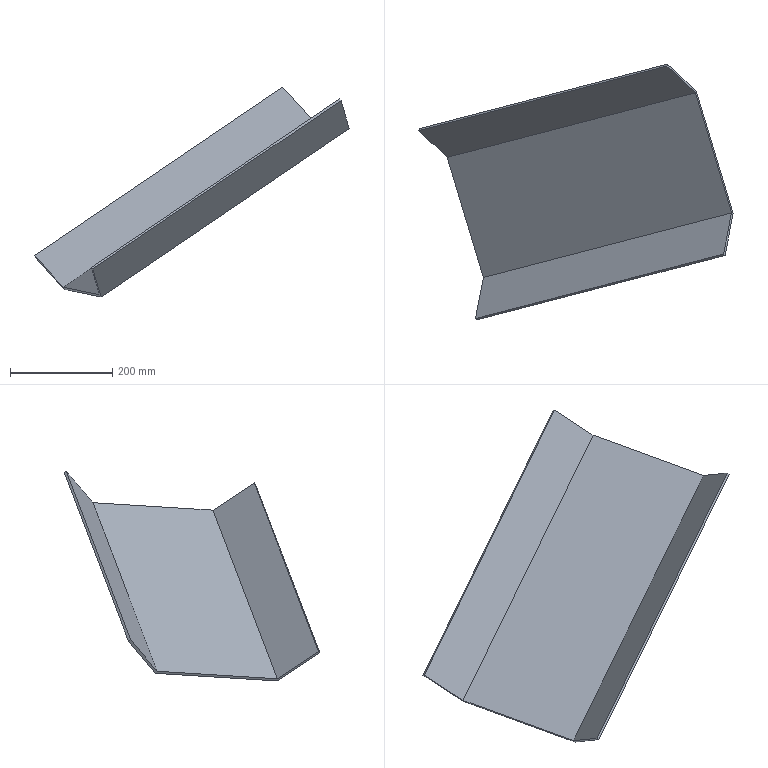Component | SolidWorks | CrusherFrameBaffle-1 | 1 solid | 10 faces | box 614.71 x 499.76 x 410.48 mm | volume 1337574 mm3 | plane 10
build123d program:
from build123d import *

# Parameters (mm, degrees)
EXTRUDE_THIN1_DEPTH = 600


with BuildPart() as part:
    # Sketch1 → Extrude-Thin1 (new body)
    with BuildSketch(Plane.XY):
        Polygon((70.711, -70.711), (0, 0), (0, 250), (70.711, 320.711), (74.246, 317.175), (5, 247.929), (5, 2.071), (74.246, -67.175), align=None)
    extrude(amount=EXTRUDE_THIN1_DEPTH)


solid = part.part

# Placed as in the assembly
solid = solid.moved(Location((-188.681, -31.644, -552.552), (-20.862, 53.982, -150.678)))
STEP:
#1=CARTESIAN_POINT('',(-4.718,-10.616,-22.172));
#2=VERTEX_POINT('',#1);
#3=CARTESIAN_POINT('',(-5.331,-13.784,-20.063));
#4=VERTEX_POINT('',#3);
#5=CARTESIAN_POINT('',(-4.705,-10.549,-22.217));
#6=DIRECTION('',(-0.1589,-0.8218,0.5471));
#7=VECTOR('',#6,39.37);
#8=LINE('',#5,#7);
#9=EDGE_CURVE('',#2,#4,#8,.T.);
#10=ORIENTED_EDGE('',*,*,#9,.T.);
#11=CARTESIAN_POINT('',(13.775,-8.838,-7.083));
#12=VERTEX_POINT('',#11);
#13=CARTESIAN_POINT('',(13.775,-8.838,-7.083));
#14=DIRECTION('',(-0.8088,-0.2094,-0.5495));
#15=VECTOR('',#14,39.37);
#16=LINE('',#13,#15);
#17=EDGE_CURVE('',#12,#4,#16,.T.);
#18=ORIENTED_EDGE('',*,*,#17,.F.);
#19=CARTESIAN_POINT('',(14.388,-5.669,-9.192));
#20=VERTEX_POINT('',#19);
#21=CARTESIAN_POINT('',(14.401,-5.602,-9.237));
#22=DIRECTION('',(-0.1589,-0.8218,0.5471));
#23=VECTOR('',#22,39.37);
#24=LINE('',#21,#23);
#25=EDGE_CURVE('',#20,#12,#24,.T.);
#26=ORIENTED_EDGE('',*,*,#25,.F.);
#27=CARTESIAN_POINT('',(14.388,-5.669,-9.192));
#28=DIRECTION('',(-0.8088,-0.2094,-0.5495));
#29=VECTOR('',#28,39.37);
#30=LINE('',#27,#29);
#31=EDGE_CURVE('',#20,#2,#30,.T.);
#32=ORIENTED_EDGE('',*,*,#31,.T.);
#33=EDGE_LOOP('',(#10,#18,#26,#32));
#34=FACE_OUTER_BOUND('',#33,.T.);
#35=CARTESIAN_POINT('',(14.401,-5.602,-9.237));
#36=DIRECTION('',(0.5662,-0.5298,-0.6315));
#37=DIRECTION('',(0.1589,0.8218,-0.5471));
#38=AXIS2_PLACEMENT_3D('',#35,#36,#37);
#39=PLANE('',#38);
#40=ADVANCED_FACE('',(#34),#39,.F.);
#41=CARTESIAN_POINT('',(-5.22,-13.889,-20.187));
#42=VERTEX_POINT('',#41);
#43=CARTESIAN_POINT('',(-5.22,-13.889,-20.187));
#44=DIRECTION('',(-0.5662,0.5298,0.6315));
#45=VECTOR('',#44,39.37);
#46=LINE('',#43,#45);
#47=EDGE_CURVE('',#42,#4,#46,.T.);
#48=ORIENTED_EDGE('',*,*,#47,.F.);
#49=CARTESIAN_POINT('',(13.887,-8.942,-7.207));
#50=VERTEX_POINT('',#49);
#51=CARTESIAN_POINT('',(13.887,-8.942,-7.207));
#52=DIRECTION('',(-0.8088,-0.2094,-0.5495));
#53=VECTOR('',#52,39.37);
#54=LINE('',#51,#53);
#55=EDGE_CURVE('',#50,#42,#54,.T.);
#56=ORIENTED_EDGE('',*,*,#55,.F.);
#57=CARTESIAN_POINT('',(13.887,-8.942,-7.207));
#58=DIRECTION('',(-0.5662,0.5298,0.6315));
#59=VECTOR('',#58,39.37);
#60=LINE('',#57,#59);
#61=EDGE_CURVE('',#50,#12,#60,.T.);
#62=ORIENTED_EDGE('',*,*,#61,.T.);
#63=ORIENTED_EDGE('',*,*,#17,.T.);
#64=EDGE_LOOP('',(#48,#56,#62,#63));
#65=FACE_OUTER_BOUND('',#64,.T.);
#66=CARTESIAN_POINT('',(13.887,-8.942,-7.207));
#67=DIRECTION('',(-0.1589,-0.8218,0.5471));
#68=DIRECTION('',(0.5662,-0.5298,-0.6315));
#69=AXIS2_PLACEMENT_3D('',#66,#67,#68);
#70=PLANE('',#69);
#71=ADVANCED_FACE('',(#65),#70,.T.);
#72=CARTESIAN_POINT('',(-4.594,-10.653,-22.341));
#73=VERTEX_POINT('',#72);
#74=CARTESIAN_POINT('',(-4.594,-10.653,-22.341));
#75=DIRECTION('',(-0.1589,-0.8218,0.5471));
#76=VECTOR('',#75,39.37);
#77=LINE('',#74,#76);
#78=EDGE_CURVE('',#73,#42,#77,.T.);
#79=ORIENTED_EDGE('',*,*,#78,.F.);
#80=CARTESIAN_POINT('',(14.512,-5.706,-9.361));
#81=VERTEX_POINT('',#80);
#82=CARTESIAN_POINT('',(14.512,-5.706,-9.361));
#83=DIRECTION('',(-0.8088,-0.2094,-0.5495));
#84=VECTOR('',#83,39.37);
#85=LINE('',#82,#84);
#86=EDGE_CURVE('',#81,#73,#85,.T.);
#87=ORIENTED_EDGE('',*,*,#86,.F.);
#88=CARTESIAN_POINT('',(14.512,-5.706,-9.361));
#89=DIRECTION('',(-0.1589,-0.8218,0.5471));
#90=VECTOR('',#89,39.37);
#91=LINE('',#88,#90);
#92=EDGE_CURVE('',#81,#50,#91,.T.);
#93=ORIENTED_EDGE('',*,*,#92,.T.);
#94=ORIENTED_EDGE('',*,*,#55,.T.);
#95=EDGE_LOOP('',(#79,#87,#93,#94));
#96=FACE_OUTER_BOUND('',#95,.T.);
#97=CARTESIAN_POINT('',(14.512,-5.706,-9.361));
#98=DIRECTION('',(0.5662,-0.5298,-0.6315));
#99=DIRECTION('',(0.1589,0.8218,-0.5471));
#100=AXIS2_PLACEMENT_3D('',#97,#98,#99);
#101=PLANE('',#100);
#102=ADVANCED_FACE('',(#96),#101,.T.);
#103=CARTESIAN_POINT('',(-7.428,-1.246,-21.754));
#104=VERTEX_POINT('',#103);
#105=CARTESIAN_POINT('',(-7.428,-1.246,-21.754));
#106=DIRECTION('',(0.288,-0.9558,-0.05964));
#107=VECTOR('',#106,39.37);
#108=LINE('',#105,#107);
#109=EDGE_CURVE('',#104,#73,#108,.T.);
#110=ORIENTED_EDGE('',*,*,#109,.F.);
#111=CARTESIAN_POINT('',(11.678,3.701,-8.774));
#112=VERTEX_POINT('',#111);
#113=CARTESIAN_POINT('',(11.678,3.701,-8.774));
#114=DIRECTION('',(-0.8088,-0.2094,-0.5495));
#115=VECTOR('',#114,39.37);
#116=LINE('',#113,#115);
#117=EDGE_CURVE('',#112,#104,#116,.T.);
#118=ORIENTED_EDGE('',*,*,#117,.F.);
#119=CARTESIAN_POINT('',(11.678,3.701,-8.774));
#120=DIRECTION('',(0.288,-0.9558,-0.05964));
#121=VECTOR('',#120,39.37);
#122=LINE('',#119,#121);
#123=EDGE_CURVE('',#112,#81,#122,.T.);
#124=ORIENTED_EDGE('',*,*,#123,.T.);
#125=ORIENTED_EDGE('',*,*,#86,.T.);
#126=EDGE_LOOP('',(#110,#118,#124,#125));
#127=FACE_OUTER_BOUND('',#126,.T.);
#128=CARTESIAN_POINT('',(11.678,3.701,-8.774));
#129=DIRECTION('',(0.5127,0.2065,-0.8334));
#130=DIRECTION('',(0.8088,0.2094,0.5495));
#131=AXIS2_PLACEMENT_3D('',#128,#129,#130);
#132=PLANE('',#131);
#133=ADVANCED_FACE('',(#127),#132,.T.);
#134=CARTESIAN_POINT('',(-9.657,0.8402,-19.268));
#135=VERTEX_POINT('',#134);
#136=CARTESIAN_POINT('',(-7.428,-1.246,-21.754));
#137=DIRECTION('',(0.5662,-0.5298,-0.6315));
#138=VECTOR('',#137,39.37);
#139=LINE('',#136,#138);
#140=EDGE_CURVE('',#135,#104,#139,.T.);
#141=ORIENTED_EDGE('',*,*,#140,.F.);
#142=CARTESIAN_POINT('',(9.449,5.787,-6.288));
#143=VERTEX_POINT('',#142);
#144=CARTESIAN_POINT('',(9.449,5.787,-6.288));
#145=DIRECTION('',(-0.8088,-0.2094,-0.5495));
#146=VECTOR('',#145,39.37);
#147=LINE('',#144,#146);
#148=EDGE_CURVE('',#143,#135,#147,.T.);
#149=ORIENTED_EDGE('',*,*,#148,.F.);
#150=CARTESIAN_POINT('',(11.678,3.701,-8.774));
#151=DIRECTION('',(0.5662,-0.5298,-0.6315));
#152=VECTOR('',#151,39.37);
#153=LINE('',#150,#152);
#154=EDGE_CURVE('',#143,#112,#153,.T.);
#155=ORIENTED_EDGE('',*,*,#154,.T.);
#156=ORIENTED_EDGE('',*,*,#117,.T.);
#157=EDGE_LOOP('',(#141,#149,#155,#156));
#158=FACE_OUTER_BOUND('',#157,.T.);
#159=CARTESIAN_POINT('',(11.678,3.701,-8.774));
#160=DIRECTION('',(0.1589,0.8218,-0.5471));
#161=DIRECTION('',(-0.5662,0.5298,0.6315));
#162=AXIS2_PLACEMENT_3D('',#159,#160,#161);
#163=PLANE('',#162);
#164=ADVANCED_FACE('',(#158),#163,.T.);
#165=CARTESIAN_POINT('',(-9.689,0.6784,-19.16));
#166=VERTEX_POINT('',#165);
#167=CARTESIAN_POINT('',(-9.689,0.6784,-19.16));
#168=DIRECTION('',(0.1589,0.8218,-0.5471));
#169=VECTOR('',#168,39.37);
#170=LINE('',#167,#169);
#171=EDGE_CURVE('',#166,#135,#170,.T.);
#172=ORIENTED_EDGE('',*,*,#171,.F.);
#173=CARTESIAN_POINT('',(9.418,5.625,-6.18));
#174=VERTEX_POINT('',#173);
#175=CARTESIAN_POINT('',(9.418,5.625,-6.18));
#176=DIRECTION('',(-0.8088,-0.2094,-0.5495));
#177=VECTOR('',#176,39.37);
#178=LINE('',#175,#177);
#179=EDGE_CURVE('',#174,#166,#178,.T.);
#180=ORIENTED_EDGE('',*,*,#179,.F.);
#181=CARTESIAN_POINT('',(9.418,5.625,-6.18));
#182=DIRECTION('',(0.1589,0.8218,-0.5471));
#183=VECTOR('',#182,39.37);
#184=LINE('',#181,#183);
#185=EDGE_CURVE('',#174,#143,#184,.T.);
#186=ORIENTED_EDGE('',*,*,#185,.T.);
#187=ORIENTED_EDGE('',*,*,#148,.T.);
#188=EDGE_LOOP('',(#172,#180,#186,#187));
#189=FACE_OUTER_BOUND('',#188,.T.);
#190=CARTESIAN_POINT('',(9.418,5.625,-6.18));
#191=DIRECTION('',(-0.5662,0.5298,0.6315));
#192=DIRECTION('',(-0.1589,-0.8218,0.5471));
#193=AXIS2_PLACEMENT_3D('',#190,#191,#192);
#194=PLANE('',#193);
#195=ADVANCED_FACE('',(#189),#194,.T.);
#196=CARTESIAN_POINT('',(-7.506,-1.364,-21.595));
#197=VERTEX_POINT('',#196);
#198=CARTESIAN_POINT('',(-7.46,-1.408,-21.646));
#199=DIRECTION('',(0.5662,-0.5298,-0.6315));
#200=VECTOR('',#199,39.37);
#201=LINE('',#198,#200);
#202=EDGE_CURVE('',#166,#197,#201,.T.);
#203=ORIENTED_EDGE('',*,*,#202,.T.);
#204=CARTESIAN_POINT('',(11.6,3.582,-8.615));
#205=VERTEX_POINT('',#204);
#206=CARTESIAN_POINT('',(11.6,3.582,-8.615));
#207=DIRECTION('',(-0.8088,-0.2094,-0.5495));
#208=VECTOR('',#207,39.37);
#209=LINE('',#206,#208);
#210=EDGE_CURVE('',#205,#197,#209,.T.);
#211=ORIENTED_EDGE('',*,*,#210,.F.);
#212=CARTESIAN_POINT('',(11.647,3.539,-8.666));
#213=DIRECTION('',(0.5662,-0.5298,-0.6315));
#214=VECTOR('',#213,39.37);
#215=LINE('',#212,#214);
#216=EDGE_CURVE('',#174,#205,#215,.T.);
#217=ORIENTED_EDGE('',*,*,#216,.F.);
#218=ORIENTED_EDGE('',*,*,#179,.T.);
#219=EDGE_LOOP('',(#203,#211,#217,#218));
#220=FACE_OUTER_BOUND('',#219,.T.);
#221=CARTESIAN_POINT('',(11.647,3.539,-8.666));
#222=DIRECTION('',(0.1589,0.8218,-0.5471));
#223=DIRECTION('',(-0.5662,0.5298,0.6315));
#224=AXIS2_PLACEMENT_3D('',#221,#222,#223);
#225=PLANE('',#224);
#226=ADVANCED_FACE('',(#220),#225,.F.);
#227=CARTESIAN_POINT('',(-7.529,-1.286,-21.59));
#228=DIRECTION('',(0.288,-0.9558,-0.05964));
#229=VECTOR('',#228,39.37);
#230=LINE('',#227,#229);
#231=EDGE_CURVE('',#197,#2,#230,.T.);
#232=ORIENTED_EDGE('',*,*,#231,.T.);
#233=ORIENTED_EDGE('',*,*,#31,.F.);
#234=CARTESIAN_POINT('',(11.577,3.66,-8.61));
#235=DIRECTION('',(0.288,-0.9558,-0.05964));
#236=VECTOR('',#235,39.37);
#237=LINE('',#234,#236);
#238=EDGE_CURVE('',#205,#20,#237,.T.);
#239=ORIENTED_EDGE('',*,*,#238,.F.);
#240=ORIENTED_EDGE('',*,*,#210,.T.);
#241=EDGE_LOOP('',(#232,#233,#239,#240));
#242=FACE_OUTER_BOUND('',#241,.T.);
#243=CARTESIAN_POINT('',(11.577,3.66,-8.61));
#244=DIRECTION('',(0.5127,0.2065,-0.8334));
#245=DIRECTION('',(0.8088,0.2094,0.5495));
#246=AXIS2_PLACEMENT_3D('',#243,#244,#245);
#247=PLANE('',#246);
#248=ADVANCED_FACE('',(#242),#247,.F.);
#249=ORIENTED_EDGE('',*,*,#25,.T.);
#250=ORIENTED_EDGE('',*,*,#61,.F.);
#251=ORIENTED_EDGE('',*,*,#92,.F.);
#252=ORIENTED_EDGE('',*,*,#123,.F.);
#253=ORIENTED_EDGE('',*,*,#154,.F.);
#254=ORIENTED_EDGE('',*,*,#185,.F.);
#255=ORIENTED_EDGE('',*,*,#216,.T.);
#256=ORIENTED_EDGE('',*,*,#238,.T.);
#257=EDGE_LOOP('',(#249,#250,#251,#252,#253,#254,#255,#256));
#258=FACE_OUTER_BOUND('',#257,.T.);
#259=CARTESIAN_POINT('',(13.775,-8.838,-7.083));
#260=DIRECTION('',(-0.8088,-0.2094,-0.5495));
#261=DIRECTION('',(0.5127,0.2065,-0.8334));
#262=AXIS2_PLACEMENT_3D('',#259,#260,#261);
#263=PLANE('',#262);
#264=ADVANCED_FACE('',(#258),#263,.F.);
#265=ORIENTED_EDGE('',*,*,#9,.F.);
#266=ORIENTED_EDGE('',*,*,#231,.F.);
#267=ORIENTED_EDGE('',*,*,#202,.F.);
#268=ORIENTED_EDGE('',*,*,#171,.T.);
#269=ORIENTED_EDGE('',*,*,#140,.T.);
#270=ORIENTED_EDGE('',*,*,#109,.T.);
#271=ORIENTED_EDGE('',*,*,#78,.T.);
#272=ORIENTED_EDGE('',*,*,#47,.T.);
#273=EDGE_LOOP('',(#265,#266,#267,#268,#269,#270,#271,#272));
#274=FACE_OUTER_BOUND('',#273,.T.);
#275=CARTESIAN_POINT('',(-5.331,-13.784,-20.063));
#276=DIRECTION('',(-0.8088,-0.2094,-0.5495));
#277=DIRECTION('',(0.5127,0.2065,-0.8334));
#278=AXIS2_PLACEMENT_3D('',#275,#276,#277);
#279=PLANE('',#278);
#280=ADVANCED_FACE('',(#274),#279,.T.);
#281=CLOSED_SHELL('',(#40,#71,#102,#133,#164,#195,#226,#248,#264,#280));
#282=MANIFOLD_SOLID_BREP('',#281);
#283=CARTESIAN_POINT('',(0.,0.,0.));
#284=DIRECTION('',(0.,0.,1.));
#285=DIRECTION('',(1.,0.,0.));
#286=AXIS2_PLACEMENT_3D('',#283,#284,#285);
#287=(LENGTH_UNIT()NAMED_UNIT(*)SI_UNIT($,.METRE.));
#288=LENGTH_MEASURE_WITH_UNIT(LENGTH_MEASURE(0.0254),#287);
#289=DIMENSIONAL_EXPONENTS(1.,0.,0.,0.,0.,0.,0.);
#290=(CONVERSION_BASED_UNIT('',#288)LENGTH_UNIT()NAMED_UNIT(#289));
#291=UNCERTAINTY_MEASURE_WITH_UNIT(LENGTH_MEASURE(0.00001),#290,'','');
#292=(NAMED_UNIT(*)PLANE_ANGLE_UNIT()SI_UNIT($,.RADIAN.));
#293=(NAMED_UNIT(*)SI_UNIT($,.STERADIAN.)SOLID_ANGLE_UNIT());
#294=(GEOMETRIC_REPRESENTATION_CONTEXT(3)GLOBAL_UNCERTAINTY_ASSIGNED_CONTEXT((#291))GLOBAL_UNIT_ASSIGNED_CONTEXT((#290,#292,#293))REPRESENTATION_CONTEXT('',''));
#295=ADVANCED_BREP_SHAPE_REPRESENTATION('',(#282,#286),#294);
#296=COLOUR_RGB('',0.7922,0.8196,0.9333);
#297=FILL_AREA_STYLE_COLOUR('',#296);
#298=FILL_AREA_STYLE('',(#297));
#299=SURFACE_STYLE_FILL_AREA(#298);
#300=SURFACE_SIDE_STYLE('',(#299));
#301=SURFACE_STYLE_USAGE(.BOTH.,#300);
#302=PRESENTATION_STYLE_ASSIGNMENT((#301));
#303=STYLED_ITEM('',(#302),#282);
#304=PRESENTATION_LAYER_ASSIGNMENT('','',(#303));
#305=(LENGTH_UNIT()NAMED_UNIT(*)SI_UNIT($,.METRE.));
#306=LENGTH_MEASURE_WITH_UNIT(LENGTH_MEASURE(0.0254),#305);
#307=DIMENSIONAL_EXPONENTS(1.,0.,0.,0.,0.,0.,0.);
#308=(CONVERSION_BASED_UNIT('',#306)LENGTH_UNIT()NAMED_UNIT(#307));
#309=UNCERTAINTY_MEASURE_WITH_UNIT(LENGTH_MEASURE(0.00001),#308,'','');
#310=(NAMED_UNIT(*)PLANE_ANGLE_UNIT()SI_UNIT($,.RADIAN.));
#311=(NAMED_UNIT(*)SI_UNIT($,.STERADIAN.)SOLID_ANGLE_UNIT());
#312=(GEOMETRIC_REPRESENTATION_CONTEXT(3)GLOBAL_UNCERTAINTY_ASSIGNED_CONTEXT((#309))GLOBAL_UNIT_ASSIGNED_CONTEXT((#308,#310,#311))REPRESENTATION_CONTEXT('',''));
#313=MECHANICAL_DESIGN_GEOMETRIC_PRESENTATION_REPRESENTATION('',(#303),#312);